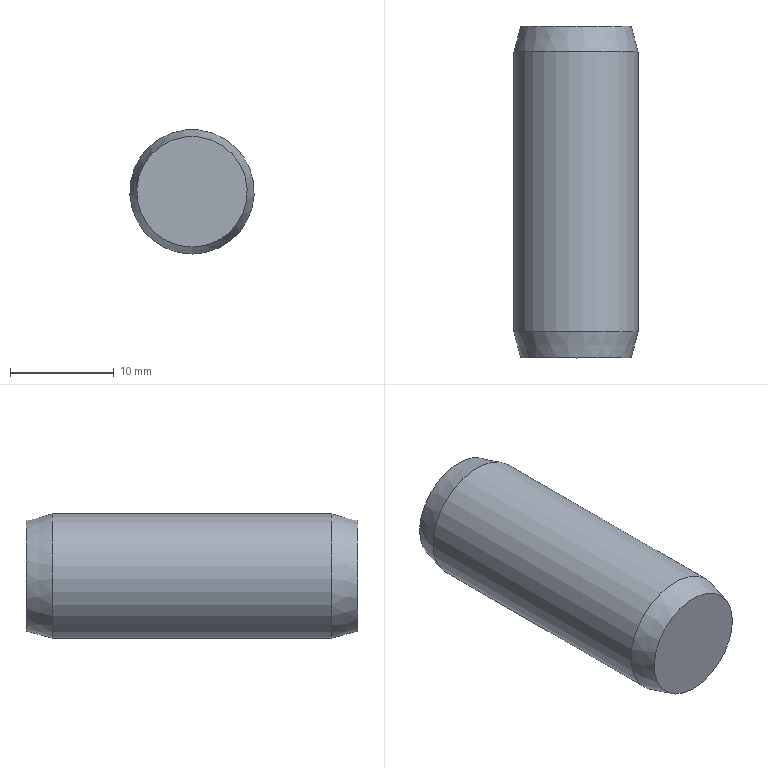Component | NX | GB-T119_1-2000_12X32 | 1 solid | 5 faces | box 12 x 32 x 12 mm | volume 3558 mm3 | plane 2 | cone 2 | cylinder 1 | commonest cylinder face diameters 12 x1
STEP:
#1=CARTESIAN_POINT('',(0.,0.,0.));
#2=DIRECTION('',(0.,0.,1.));
#3=DIRECTION('',(1.,0.,0.));
#4=AXIS2_PLACEMENT_3D('',#1,#2,#3);
#5=CARTESIAN_POINT('',(30.,-26.,35.67));
#6=VERTEX_POINT('',#5);
#7=CARTESIAN_POINT('',(30.,-26.,41.));
#8=DIRECTION('',(0.,1.,0.));
#9=DIRECTION('',(0.,0.,-1.));
#10=AXIS2_PLACEMENT_3D('',#7,#8,#9);
#11=CIRCLE('',#10,5.33);
#12=CARTESIAN_POINT('',(30.,-26.,41.));
#13=DIRECTION('',(0.,1.,0.));
#14=DIRECTION('',(0.,0.,-1.));
#15=AXIS2_PLACEMENT_3D('',#12,#13,#14);
#16=PLANE('',#15);
#17=CARTESIAN_POINT('',(0.,0.));
#18=DIRECTION('',(1.,0.));
#19=AXIS2_PLACEMENT_2D('',#17,#18);
#20=CIRCLE('',#19,5.33);
#21=(GEOMETRIC_REPRESENTATION_CONTEXT(2)PARAMETRIC_REPRESENTATION_CONTEXT()REPRESENTATION_CONTEXT('',''));
#22=DEFINITIONAL_REPRESENTATION('',(#20),#21);
#23=PCURVE('',#16,#22);
#24=CARTESIAN_POINT('',(30.,-26.,41.));
#25=DIRECTION('',(0.,-1.,0.));
#26=DIRECTION('',(0.,0.,1.));
#27=AXIS2_PLACEMENT_3D('',#24,#25,#26);
#28=CONICAL_SURFACE('',#27,5.33,0.2618);
#29=CARTESIAN_POINT('',(9.425,-0.));
#30=DIRECTION('',(-1.,0.));
#31=VECTOR('',#30,1.);
#32=LINE('',#29,#31);
#33=(GEOMETRIC_REPRESENTATION_CONTEXT(2)PARAMETRIC_REPRESENTATION_CONTEXT()REPRESENTATION_CONTEXT('',''));
#34=DEFINITIONAL_REPRESENTATION('',(#32),#33);
#35=PCURVE('',#28,#34);
#36=SURFACE_CURVE('',#11,(#23,#35),.PCURVE_S1.);
#37=EDGE_CURVE('',#6,#6,#36,.T.);
#38=ORIENTED_EDGE('',*,*,#37,.T.);
#39=EDGE_LOOP('',(#38));
#40=FACE_BOUND('',#39,.T.);
#41=ADVANCED_FACE('',(#40),#16,.T.);
#42=CARTESIAN_POINT('',(30.,-28.5,35.));
#43=VERTEX_POINT('',#42);
#44=CARTESIAN_POINT('',(30.,-28.5,41.));
#45=DIRECTION('',(0.,1.,0.));
#46=DIRECTION('',(0.,0.,-1.));
#47=AXIS2_PLACEMENT_3D('',#44,#45,#46);
#48=CIRCLE('',#47,6.);
#49=CARTESIAN_POINT('',(9.425,2.5));
#50=DIRECTION('',(-1.,0.));
#51=VECTOR('',#50,1.);
#52=LINE('',#49,#51);
#53=(GEOMETRIC_REPRESENTATION_CONTEXT(2)PARAMETRIC_REPRESENTATION_CONTEXT()REPRESENTATION_CONTEXT('',''));
#54=DEFINITIONAL_REPRESENTATION('',(#52),#53);
#55=PCURVE('',#28,#54);
#56=CARTESIAN_POINT('',(30.,-58.,41.));
#57=DIRECTION('',(0.,1.,0.));
#58=DIRECTION('',(0.,0.,-1.));
#59=AXIS2_PLACEMENT_3D('',#56,#57,#58);
#60=CYLINDRICAL_SURFACE('',#59,6.);
#61=CARTESIAN_POINT('',(0.,29.5));
#62=DIRECTION('',(1.,0.));
#63=VECTOR('',#62,1.);
#64=LINE('',#61,#63);
#65=(GEOMETRIC_REPRESENTATION_CONTEXT(2)PARAMETRIC_REPRESENTATION_CONTEXT()REPRESENTATION_CONTEXT('',''));
#66=DEFINITIONAL_REPRESENTATION('',(#64),#65);
#67=PCURVE('',#60,#66);
#68=SURFACE_CURVE('',#48,(#55,#67),.PCURVE_S1.);
#69=EDGE_CURVE('',#43,#43,#68,.T.);
#70=ORIENTED_EDGE('',*,*,#69,.T.);
#71=CARTESIAN_POINT('',(30.,-26.,35.67));
#72=CARTESIAN_POINT('',(30.,-28.5,35.));
#73=B_SPLINE_CURVE_WITH_KNOTS('',1,(#71,#72),.UNSPECIFIED.,.F.,.F.,(2,2),(-0.,2.588),.PIECEWISE_BEZIER_KNOTS.);
#74=CARTESIAN_POINT('',(3.142,0.));
#75=DIRECTION('',(0.,1.));
#76=VECTOR('',#75,1.);
#77=LINE('',#74,#76);
#78=(GEOMETRIC_REPRESENTATION_CONTEXT(2)PARAMETRIC_REPRESENTATION_CONTEXT()REPRESENTATION_CONTEXT('',''));
#79=DEFINITIONAL_REPRESENTATION('',(#77),#78);
#80=PCURVE('',#28,#79);
#81=CARTESIAN_POINT('',(9.425,0.));
#82=DIRECTION('',(0.,1.));
#83=VECTOR('',#82,1.);
#84=LINE('',#81,#83);
#85=(GEOMETRIC_REPRESENTATION_CONTEXT(2)PARAMETRIC_REPRESENTATION_CONTEXT()REPRESENTATION_CONTEXT('',''));
#86=DEFINITIONAL_REPRESENTATION('',(#84),#85);
#87=PCURVE('',#28,#86);
#88=SEAM_CURVE('',#73,(#80,#87),.PCURVE_S1.);
#89=EDGE_CURVE('',#6,#43,#88,.T.);
#90=ORIENTED_EDGE('',*,*,#89,.F.);
#91=ORIENTED_EDGE('',*,*,#37,.F.);
#92=ORIENTED_EDGE('',*,*,#89,.T.);
#93=EDGE_LOOP('',(#70,#90,#91,#92));
#94=FACE_BOUND('',#93,.T.);
#95=ADVANCED_FACE('',(#94),#28,.T.);
#96=CARTESIAN_POINT('',(30.,-55.5,35.));
#97=VERTEX_POINT('',#96);
#98=CARTESIAN_POINT('',(30.,-55.5,41.));
#99=DIRECTION('',(0.,1.,0.));
#100=DIRECTION('',(0.,0.,-1.));
#101=AXIS2_PLACEMENT_3D('',#98,#99,#100);
#102=CIRCLE('',#101,6.);
#103=CARTESIAN_POINT('',(0.,2.5));
#104=DIRECTION('',(1.,0.));
#105=VECTOR('',#104,1.);
#106=LINE('',#103,#105);
#107=(GEOMETRIC_REPRESENTATION_CONTEXT(2)PARAMETRIC_REPRESENTATION_CONTEXT()REPRESENTATION_CONTEXT('',''));
#108=DEFINITIONAL_REPRESENTATION('',(#106),#107);
#109=PCURVE('',#60,#108);
#110=CARTESIAN_POINT('',(30.,-55.5,41.));
#111=DIRECTION('',(0.,1.,0.));
#112=DIRECTION('',(0.,0.,-1.));
#113=AXIS2_PLACEMENT_3D('',#110,#111,#112);
#114=CONICAL_SURFACE('',#113,6.,0.2618);
#115=CARTESIAN_POINT('',(0.,-0.));
#116=DIRECTION('',(1.,0.));
#117=VECTOR('',#116,1.);
#118=LINE('',#115,#117);
#119=(GEOMETRIC_REPRESENTATION_CONTEXT(2)PARAMETRIC_REPRESENTATION_CONTEXT()REPRESENTATION_CONTEXT('',''));
#120=DEFINITIONAL_REPRESENTATION('',(#118),#119);
#121=PCURVE('',#114,#120);
#122=SURFACE_CURVE('',#102,(#109,#121),.PCURVE_S1.);
#123=EDGE_CURVE('',#97,#97,#122,.T.);
#124=ORIENTED_EDGE('',*,*,#123,.T.);
#125=CARTESIAN_POINT('',(30.,-55.5,35.));
#126=CARTESIAN_POINT('',(30.,-28.5,35.));
#127=B_SPLINE_CURVE_WITH_KNOTS('',1,(#125,#126),.UNSPECIFIED.,.F.,.F.,(2,2),(2.5,29.5),.PIECEWISE_BEZIER_KNOTS.);
#128=CARTESIAN_POINT('',(6.283,0.));
#129=DIRECTION('',(0.,1.));
#130=VECTOR('',#129,1.);
#131=LINE('',#128,#130);
#132=(GEOMETRIC_REPRESENTATION_CONTEXT(2)PARAMETRIC_REPRESENTATION_CONTEXT()REPRESENTATION_CONTEXT('',''));
#133=DEFINITIONAL_REPRESENTATION('',(#131),#132);
#134=PCURVE('',#60,#133);
#135=CARTESIAN_POINT('',(0.,0.));
#136=DIRECTION('',(0.,1.));
#137=VECTOR('',#136,1.);
#138=LINE('',#135,#137);
#139=(GEOMETRIC_REPRESENTATION_CONTEXT(2)PARAMETRIC_REPRESENTATION_CONTEXT()REPRESENTATION_CONTEXT('',''));
#140=DEFINITIONAL_REPRESENTATION('',(#138),#139);
#141=PCURVE('',#60,#140);
#142=SEAM_CURVE('',#127,(#134,#141),.PCURVE_S1.);
#143=EDGE_CURVE('',#97,#43,#142,.T.);
#144=ORIENTED_EDGE('',*,*,#143,.T.);
#145=ORIENTED_EDGE('',*,*,#69,.F.);
#146=ORIENTED_EDGE('',*,*,#143,.F.);
#147=EDGE_LOOP('',(#124,#144,#145,#146));
#148=FACE_BOUND('',#147,.T.);
#149=ADVANCED_FACE('',(#148),#60,.T.);
#150=CARTESIAN_POINT('',(30.,-58.,35.67));
#151=VERTEX_POINT('',#150);
#152=CARTESIAN_POINT('',(30.,-58.,41.));
#153=DIRECTION('',(0.,1.,0.));
#154=DIRECTION('',(0.,0.,-1.));
#155=AXIS2_PLACEMENT_3D('',#152,#153,#154);
#156=CIRCLE('',#155,5.33);
#157=CARTESIAN_POINT('',(0.,-2.5));
#158=DIRECTION('',(1.,0.));
#159=VECTOR('',#158,1.);
#160=LINE('',#157,#159);
#161=(GEOMETRIC_REPRESENTATION_CONTEXT(2)PARAMETRIC_REPRESENTATION_CONTEXT()REPRESENTATION_CONTEXT('',''));
#162=DEFINITIONAL_REPRESENTATION('',(#160),#161);
#163=PCURVE('',#114,#162);
#164=CARTESIAN_POINT('',(30.,-58.,46.33));
#165=DIRECTION('',(0.,-1.,0.));
#166=DIRECTION('',(0.,0.,1.));
#167=AXIS2_PLACEMENT_3D('',#164,#165,#166);
#168=PLANE('',#167);
#169=CARTESIAN_POINT('',(-10.66,0.));
#170=CARTESIAN_POINT('',(-10.66,9.232));
#171=CARTESIAN_POINT('',(-2.665,4.616));
#172=CARTESIAN_POINT('',(5.33,0.));
#173=CARTESIAN_POINT('',(-2.665,-4.616));
#174=CARTESIAN_POINT('',(-10.66,-9.232));
#175=CARTESIAN_POINT('',(-10.66,0.));
#176=(BOUNDED_CURVE()B_SPLINE_CURVE(2,(#169,#170,#171,#172,#173,#174,#175),.UNSPECIFIED.,.T.,.F.)B_SPLINE_CURVE_WITH_KNOTS((1,2,2,2,2,1),(-2.094,0.,2.094,4.189,6.283,8.378),.UNSPECIFIED.)CURVE()GEOMETRIC_REPRESENTATION_ITEM()RATIONAL_B_SPLINE_CURVE((1.,0.5,1.,0.5,1.,0.5,1.))REPRESENTATION_ITEM(''));
#177=(GEOMETRIC_REPRESENTATION_CONTEXT(2)PARAMETRIC_REPRESENTATION_CONTEXT()REPRESENTATION_CONTEXT('',''));
#178=DEFINITIONAL_REPRESENTATION('',(#176),#177);
#179=PCURVE('',#168,#178);
#180=SURFACE_CURVE('',#156,(#163,#179),.PCURVE_S1.);
#181=EDGE_CURVE('',#151,#151,#180,.T.);
#182=ORIENTED_EDGE('',*,*,#181,.T.);
#183=CARTESIAN_POINT('',(30.,-58.,35.67));
#184=CARTESIAN_POINT('',(30.,-55.5,35.));
#185=B_SPLINE_CURVE_WITH_KNOTS('',1,(#183,#184),.UNSPECIFIED.,.F.,.F.,(2,2),(-2.588,-0.),.PIECEWISE_BEZIER_KNOTS.);
#186=CARTESIAN_POINT('',(6.283,0.));
#187=DIRECTION('',(0.,1.));
#188=VECTOR('',#187,1.);
#189=LINE('',#186,#188);
#190=(GEOMETRIC_REPRESENTATION_CONTEXT(2)PARAMETRIC_REPRESENTATION_CONTEXT()REPRESENTATION_CONTEXT('',''));
#191=DEFINITIONAL_REPRESENTATION('',(#189),#190);
#192=PCURVE('',#114,#191);
#193=CARTESIAN_POINT('',(0.,0.));
#194=DIRECTION('',(0.,1.));
#195=VECTOR('',#194,1.);
#196=LINE('',#193,#195);
#197=(GEOMETRIC_REPRESENTATION_CONTEXT(2)PARAMETRIC_REPRESENTATION_CONTEXT()REPRESENTATION_CONTEXT('',''));
#198=DEFINITIONAL_REPRESENTATION('',(#196),#197);
#199=PCURVE('',#114,#198);
#200=SEAM_CURVE('',#185,(#192,#199),.PCURVE_S1.);
#201=EDGE_CURVE('',#151,#97,#200,.T.);
#202=ORIENTED_EDGE('',*,*,#201,.T.);
#203=ORIENTED_EDGE('',*,*,#123,.F.);
#204=ORIENTED_EDGE('',*,*,#201,.F.);
#205=EDGE_LOOP('',(#182,#202,#203,#204));
#206=FACE_BOUND('',#205,.T.);
#207=ADVANCED_FACE('',(#206),#114,.T.);
#208=ORIENTED_EDGE('',*,*,#181,.F.);
#209=EDGE_LOOP('',(#208));
#210=FACE_BOUND('',#209,.T.);
#211=ADVANCED_FACE('',(#210),#168,.T.);
#212=CLOSED_SHELL('',(#41,#95,#149,#207,#211));
#213=MANIFOLD_SOLID_BREP('',#212);
#214=(LENGTH_UNIT()NAMED_UNIT(*)SI_UNIT(.MILLI.,.METRE.));
#215=UNCERTAINTY_MEASURE_WITH_UNIT(LENGTH_MEASURE(0.00001),#214,'','');
#216=(NAMED_UNIT(*)PLANE_ANGLE_UNIT()SI_UNIT($,.RADIAN.));
#217=(NAMED_UNIT(*)SI_UNIT($,.STERADIAN.)SOLID_ANGLE_UNIT());
#218=(GEOMETRIC_REPRESENTATION_CONTEXT(3)GLOBAL_UNCERTAINTY_ASSIGNED_CONTEXT((#215))GLOBAL_UNIT_ASSIGNED_CONTEXT((#214,#216,#217))REPRESENTATION_CONTEXT('',''));
#219=ADVANCED_BREP_SHAPE_REPRESENTATION('',(#4,#213),#218);